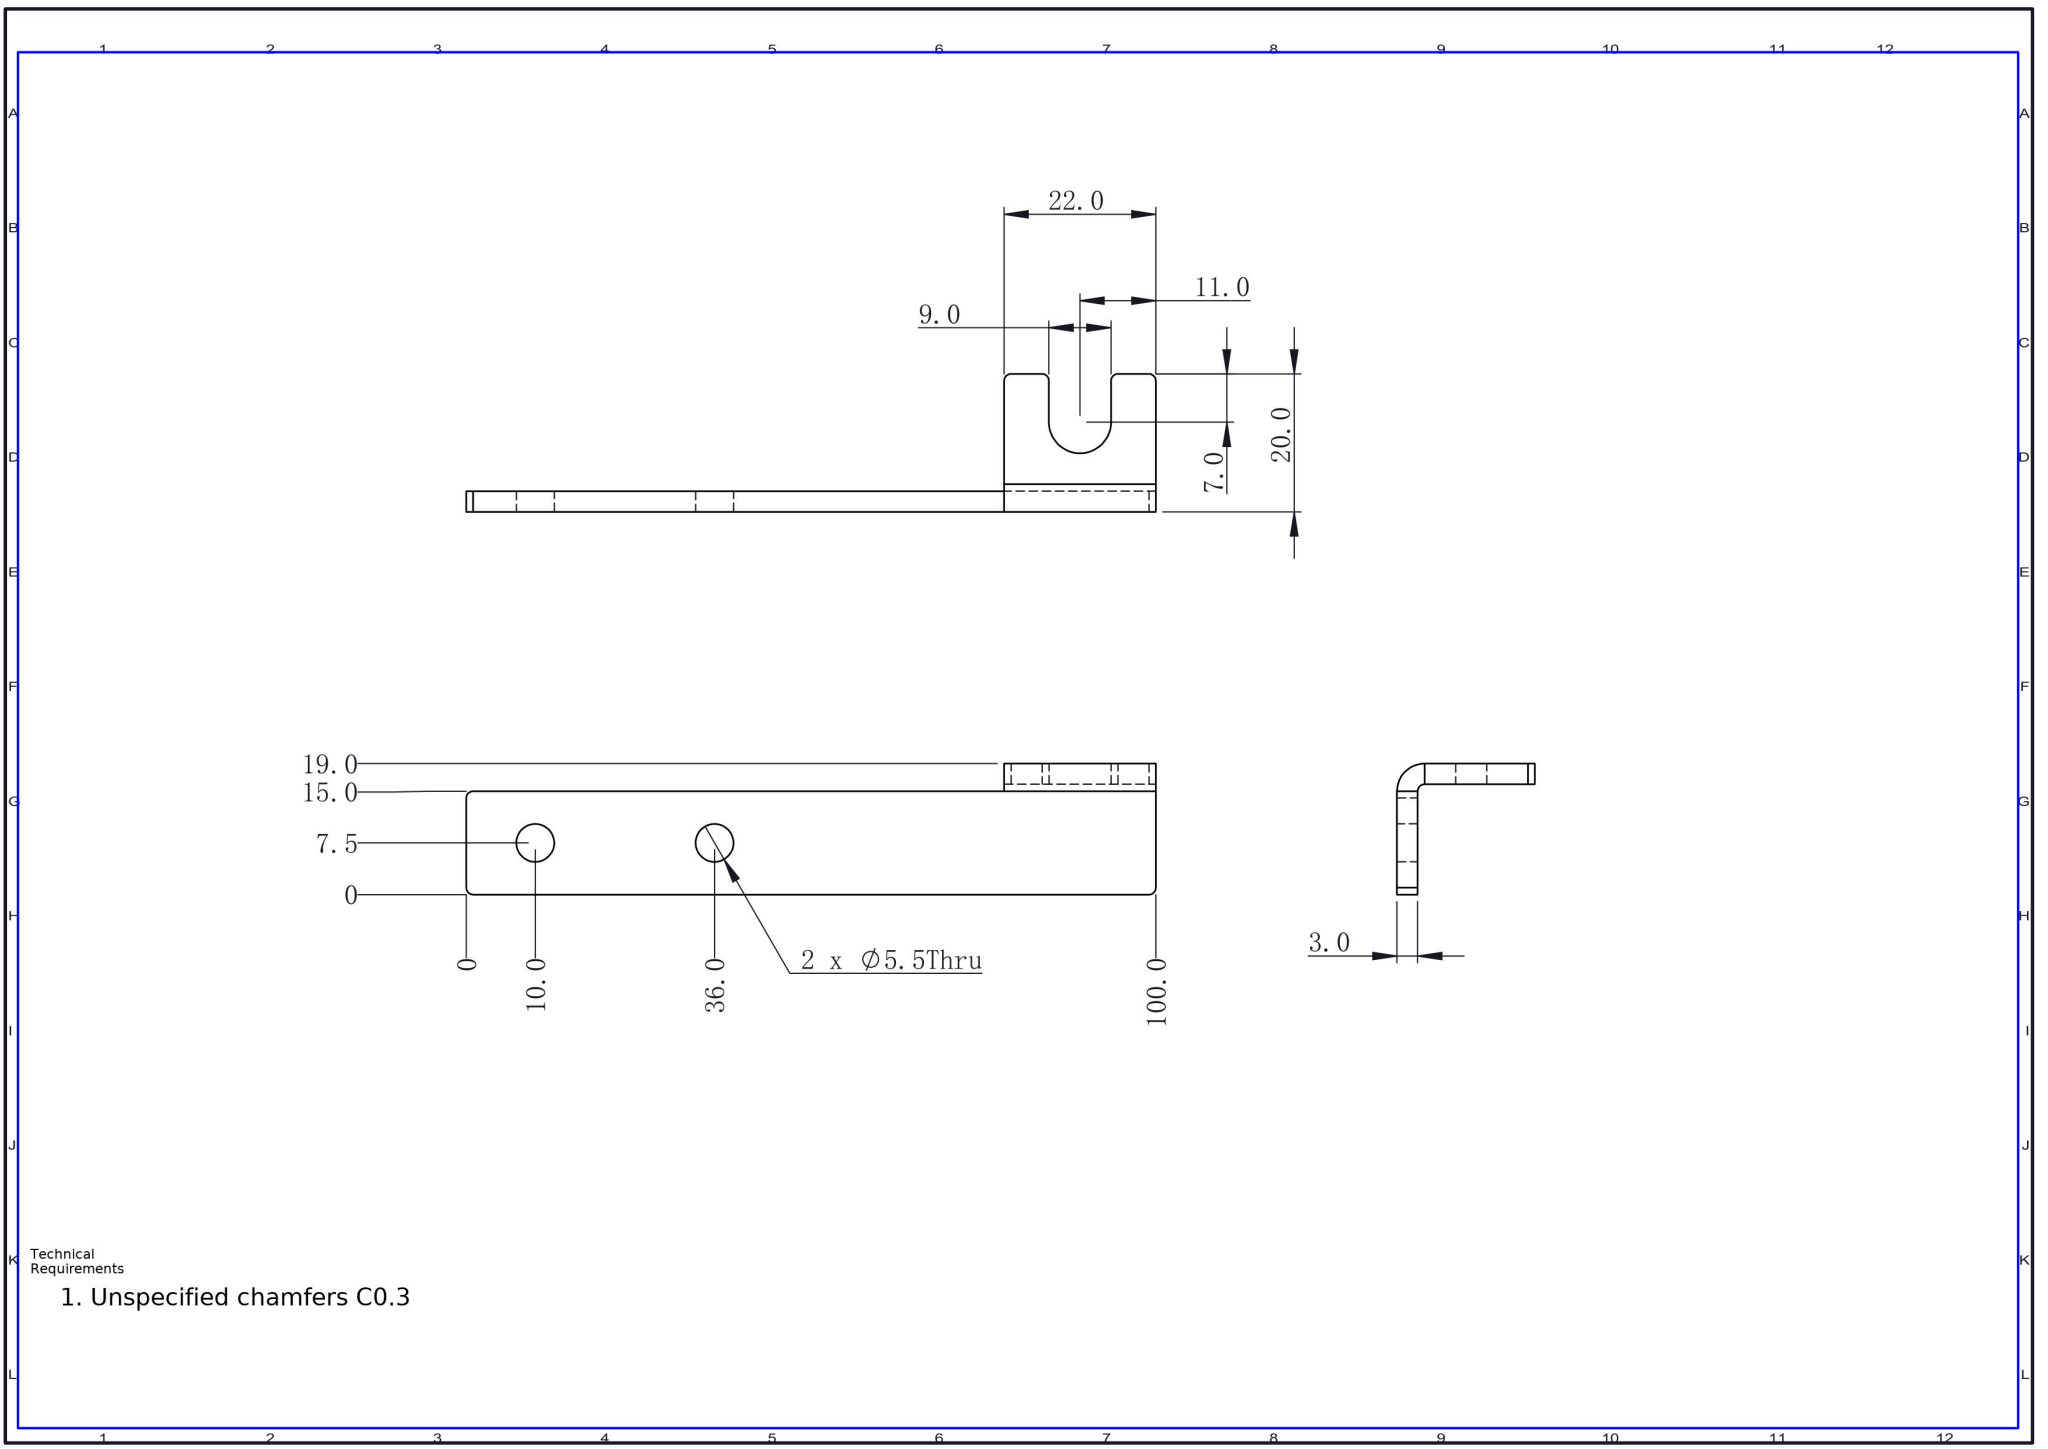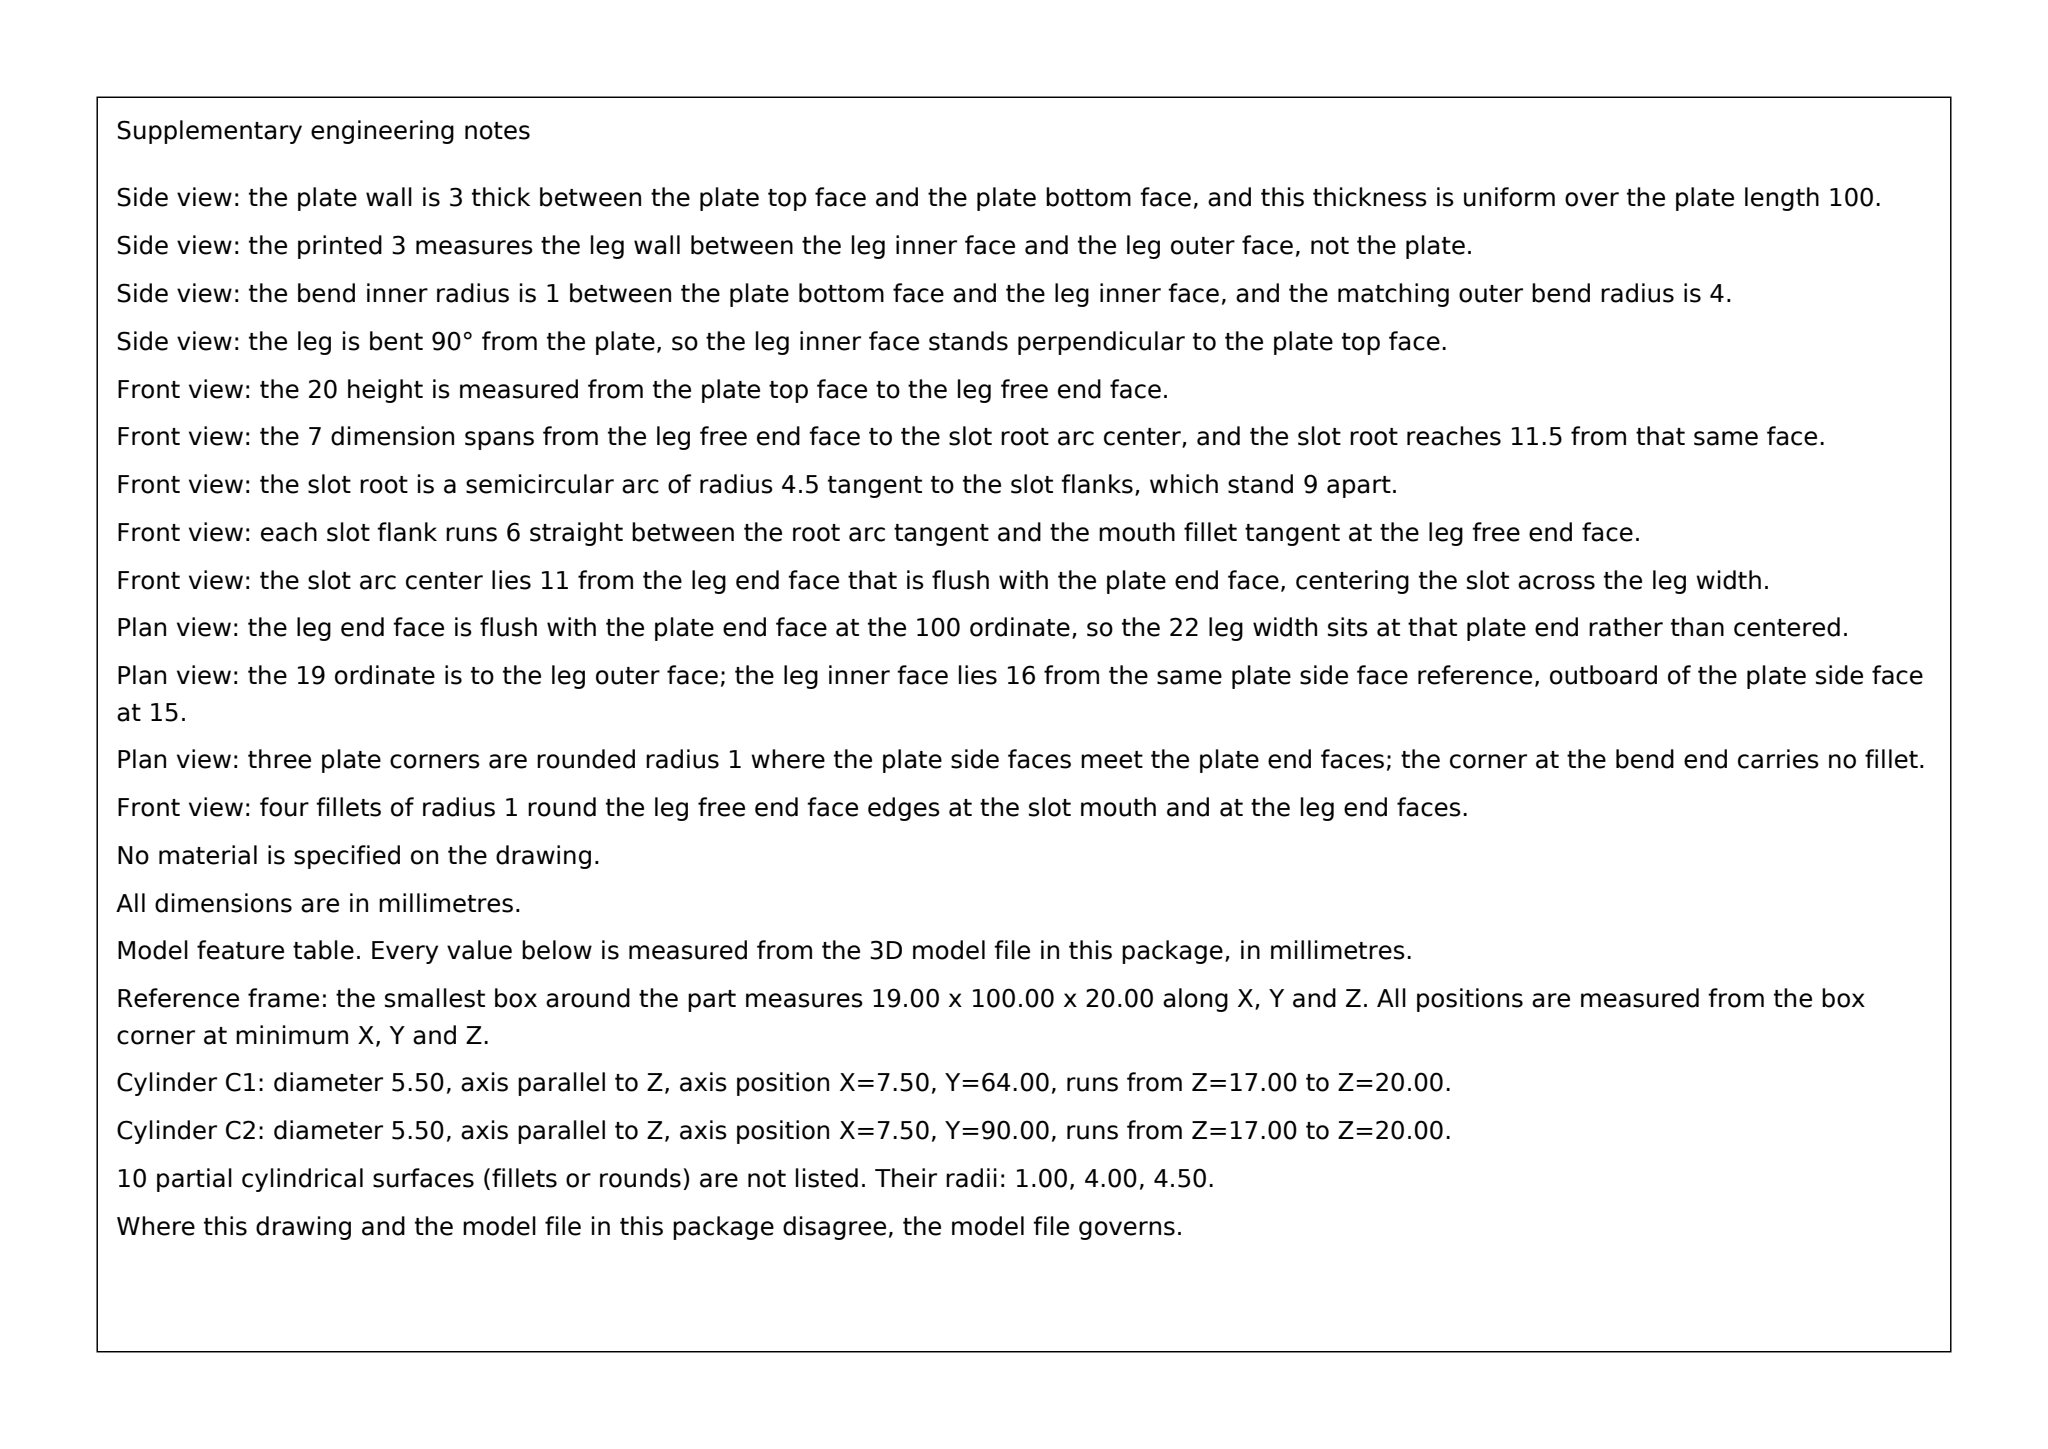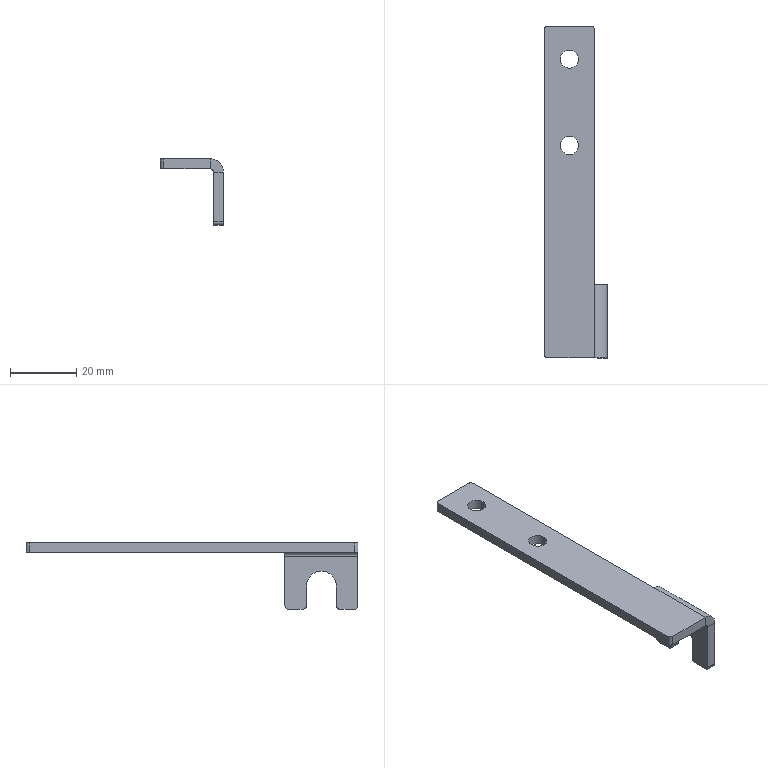Part | SolidWorks | mm | 1 solid | 30 faces | box 19 x 100 x 20 mm | volume 5384 mm3 | plane 16 | cylinder 14 | commonest cylinder face diameters 2 x8 5.5 x4 8 x1 9 x1
Drawing notes:
2X Ø5.5 THRU; hole centers 10.0 and 36.0 from the 0 end datum along the 100.0 length, 7.5 from the long edge | from the solid: cylinders 5.5 dia, axis z, pos [7.5, 90.0] and [7.5, 64.0], length 3.0 (100.0 bbox length → 10.0 and 36.0 from datum end)
Fillet balloon callouts: 3X R1.0 on base plate outline, 4X R1.0 on slot/upstand, R1.0 at bend inner corner (balloon numbers removed as illegible) | from the solid: cylinders of 2.0 dia (R1.0) along x at y/z = (1.0,1.0),(5.5,1.0),(16.5,1.0),(21.0,1.0) and along z at (1.0,1.0),(1.0,99.0),(14.0,99.0)
ALL DIMENSIONS IN MILLIMETERS | from the solid: STEP model units stated in mm; bbox_xyz 19.0 x 100.0 x 20.0 mm